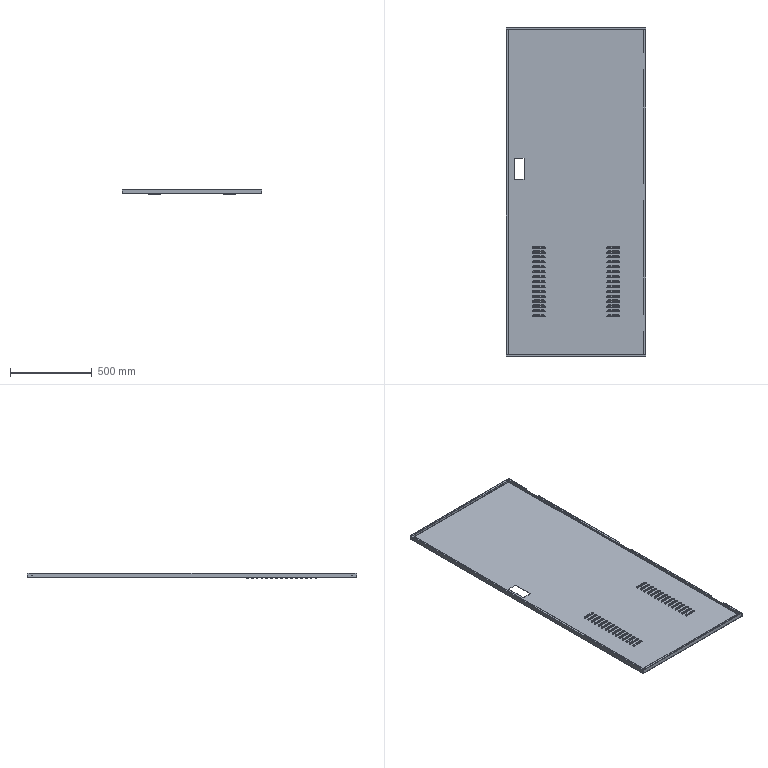Component | SolidWorks | SmallDoorPanel1-1 | 1 solid | 862 faces | volume 2872613 mm3 | cylinder 386 | torus 240 | plane 236 | commonest cylinder face diameters 8 x180 5 x90 11 x90 3.4 x13 0.4 x13